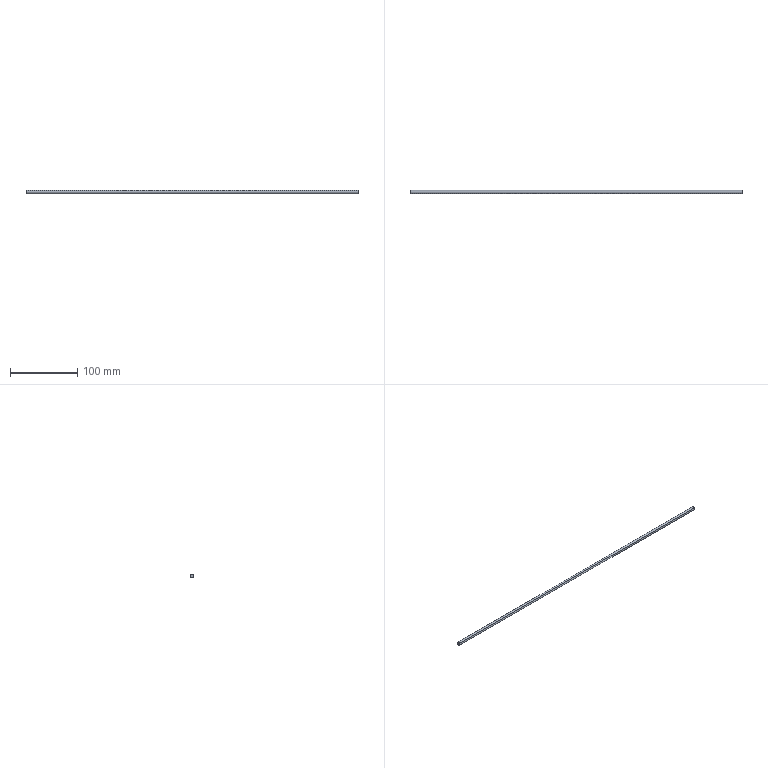Component | SolidWorks | SlideRod-2 | 1 solid | 4 faces | box 493.5 x 5 x 5 mm | volume 9690 mm3 | cylinder 2 | plane 2 | commonest cylinder face diameters 5 x2
build123d program:
from build123d import *

# Parameters (mm, degrees)
SKETCH1_R           = 2.5
BOSS_EXTRUDE1_DEPTH = 493.5


with BuildPart() as part:
    # Sketch1 → Boss-Extrude1 (new body)
    with BuildSketch(Plane(origin=(0, 0, 0), x_dir=(1, 0, 0), z_dir=(0, 1, 0))):
        with Locations(Location((0, 0, 0), (0, 0, 270))):
            Circle(SKETCH1_R)
    extrude(amount=BOSS_EXTRUDE1_DEPTH)


solid = part.part

# Placed as in the assembly
solid = solid.moved(Location((298.5, 220, -145), (0, 0, 90)))
STEP:
#1=CARTESIAN_POINT('',(11.752,8.735,-5.774));
#2=VERTEX_POINT('',#1);
#3=CARTESIAN_POINT('',(11.752,8.588,-5.643));
#4=VERTEX_POINT('',#3);
#5=CARTESIAN_POINT('',(11.752,8.661,-5.709));
#6=DIRECTION('',(1.,0.,0.));
#7=DIRECTION('',(0.,0.7491,-0.6624));
#8=AXIS2_PLACEMENT_3D('',#5,#6,#7);
#9=CIRCLE('',#8,0.09843);
#10=EDGE_CURVE('',#2,#4,#9,.T.);
#11=ORIENTED_EDGE('',*,*,#10,.F.);
#12=CARTESIAN_POINT('',(-7.677,8.735,-5.774));
#13=VERTEX_POINT('',#12);
#14=CARTESIAN_POINT('',(11.752,8.735,-5.774));
#15=DIRECTION('',(-1.,-0.,-0.));
#16=VECTOR('',#15,39.37);
#17=LINE('',#14,#16);
#18=EDGE_CURVE('',#2,#13,#17,.T.);
#19=ORIENTED_EDGE('',*,*,#18,.T.);
#20=CARTESIAN_POINT('',(-7.677,8.588,-5.643));
#21=VERTEX_POINT('',#20);
#22=CARTESIAN_POINT('',(-7.677,8.661,-5.709));
#23=DIRECTION('',(1.,0.,0.));
#24=DIRECTION('',(0.,0.7491,-0.6624));
#25=AXIS2_PLACEMENT_3D('',#22,#23,#24);
#26=CIRCLE('',#25,0.09843);
#27=EDGE_CURVE('',#13,#21,#26,.T.);
#28=ORIENTED_EDGE('',*,*,#27,.T.);
#29=CARTESIAN_POINT('',(11.752,8.588,-5.643));
#30=DIRECTION('',(-1.,-0.,-0.));
#31=VECTOR('',#30,39.37);
#32=LINE('',#29,#31);
#33=EDGE_CURVE('',#4,#21,#32,.T.);
#34=ORIENTED_EDGE('',*,*,#33,.F.);
#35=EDGE_LOOP('',(#11,#19,#28,#34));
#36=FACE_OUTER_BOUND('',#35,.T.);
#37=CARTESIAN_POINT('',(11.752,8.661,-5.709));
#38=DIRECTION('',(-1.,-0.,-0.));
#39=DIRECTION('',(0.,-0.7491,0.6624));
#40=AXIS2_PLACEMENT_3D('',#37,#38,#39);
#41=CYLINDRICAL_SURFACE('',#40,0.09843);
#42=ADVANCED_FACE('',(#36),#41,.T.);
#43=ORIENTED_EDGE('',*,*,#18,.F.);
#44=CARTESIAN_POINT('',(11.752,8.661,-5.709));
#45=DIRECTION('',(1.,0.,0.));
#46=DIRECTION('',(0.,0.7491,-0.6624));
#47=AXIS2_PLACEMENT_3D('',#44,#45,#46);
#48=CIRCLE('',#47,0.09843);
#49=EDGE_CURVE('',#4,#2,#48,.T.);
#50=ORIENTED_EDGE('',*,*,#49,.F.);
#51=ORIENTED_EDGE('',*,*,#33,.T.);
#52=CARTESIAN_POINT('',(-7.677,8.661,-5.709));
#53=DIRECTION('',(1.,0.,0.));
#54=DIRECTION('',(0.,0.7491,-0.6624));
#55=AXIS2_PLACEMENT_3D('',#52,#53,#54);
#56=CIRCLE('',#55,0.09843);
#57=EDGE_CURVE('',#21,#13,#56,.T.);
#58=ORIENTED_EDGE('',*,*,#57,.T.);
#59=EDGE_LOOP('',(#43,#50,#51,#58));
#60=FACE_OUTER_BOUND('',#59,.T.);
#61=CARTESIAN_POINT('',(11.752,8.661,-5.709));
#62=DIRECTION('',(-1.,-0.,-0.));
#63=DIRECTION('',(0.,-0.7491,0.6624));
#64=AXIS2_PLACEMENT_3D('',#61,#62,#63);
#65=CYLINDRICAL_SURFACE('',#64,0.09843);
#66=ADVANCED_FACE('',(#60),#65,.T.);
#67=ORIENTED_EDGE('',*,*,#49,.T.);
#68=ORIENTED_EDGE('',*,*,#10,.T.);
#69=EDGE_LOOP('',(#67,#68));
#70=FACE_OUTER_BOUND('',#69,.T.);
#71=CARTESIAN_POINT('',(11.752,8.661,-5.709));
#72=DIRECTION('',(1.,0.,0.));
#73=DIRECTION('',(-0.,0.7491,-0.6624));
#74=AXIS2_PLACEMENT_3D('',#71,#72,#73);
#75=PLANE('',#74);
#76=ADVANCED_FACE('',(#70),#75,.T.);
#77=ORIENTED_EDGE('',*,*,#57,.F.);
#78=ORIENTED_EDGE('',*,*,#27,.F.);
#79=EDGE_LOOP('',(#77,#78));
#80=FACE_OUTER_BOUND('',#79,.T.);
#81=CARTESIAN_POINT('',(-7.677,8.661,-5.709));
#82=DIRECTION('',(1.,0.,0.));
#83=DIRECTION('',(-0.,0.7491,-0.6624));
#84=AXIS2_PLACEMENT_3D('',#81,#82,#83);
#85=PLANE('',#84);
#86=ADVANCED_FACE('',(#80),#85,.F.);
#87=CLOSED_SHELL('',(#42,#66,#76,#86));
#88=MANIFOLD_SOLID_BREP('',#87);
#89=CARTESIAN_POINT('',(0.,0.,0.));
#90=DIRECTION('',(0.,0.,1.));
#91=DIRECTION('',(1.,0.,0.));
#92=AXIS2_PLACEMENT_3D('',#89,#90,#91);
#93=(LENGTH_UNIT()NAMED_UNIT(*)SI_UNIT($,.METRE.));
#94=LENGTH_MEASURE_WITH_UNIT(LENGTH_MEASURE(0.0254),#93);
#95=DIMENSIONAL_EXPONENTS(1.,0.,0.,0.,0.,0.,0.);
#96=(CONVERSION_BASED_UNIT('',#94)LENGTH_UNIT()NAMED_UNIT(#95));
#97=UNCERTAINTY_MEASURE_WITH_UNIT(LENGTH_MEASURE(0.00001),#96,'','');
#98=(NAMED_UNIT(*)PLANE_ANGLE_UNIT()SI_UNIT($,.RADIAN.));
#99=(NAMED_UNIT(*)SI_UNIT($,.STERADIAN.)SOLID_ANGLE_UNIT());
#100=(GEOMETRIC_REPRESENTATION_CONTEXT(3)GLOBAL_UNCERTAINTY_ASSIGNED_CONTEXT((#97))GLOBAL_UNIT_ASSIGNED_CONTEXT((#96,#98,#99))REPRESENTATION_CONTEXT('',''));
#101=ADVANCED_BREP_SHAPE_REPRESENTATION('',(#88,#92),#100);
#102=COLOUR_RGB('',0.7922,0.8196,0.9333);
#103=FILL_AREA_STYLE_COLOUR('',#102);
#104=FILL_AREA_STYLE('',(#103));
#105=SURFACE_STYLE_FILL_AREA(#104);
#106=SURFACE_SIDE_STYLE('',(#105));
#107=SURFACE_STYLE_USAGE(.BOTH.,#106);
#108=PRESENTATION_STYLE_ASSIGNMENT((#107));
#109=STYLED_ITEM('',(#108),#88);
#110=PRESENTATION_LAYER_ASSIGNMENT('','',(#109));
#111=(LENGTH_UNIT()NAMED_UNIT(*)SI_UNIT($,.METRE.));
#112=LENGTH_MEASURE_WITH_UNIT(LENGTH_MEASURE(0.0254),#111);
#113=DIMENSIONAL_EXPONENTS(1.,0.,0.,0.,0.,0.,0.);
#114=(CONVERSION_BASED_UNIT('',#112)LENGTH_UNIT()NAMED_UNIT(#113));
#115=UNCERTAINTY_MEASURE_WITH_UNIT(LENGTH_MEASURE(0.00001),#114,'','');
#116=(NAMED_UNIT(*)PLANE_ANGLE_UNIT()SI_UNIT($,.RADIAN.));
#117=(NAMED_UNIT(*)SI_UNIT($,.STERADIAN.)SOLID_ANGLE_UNIT());
#118=(GEOMETRIC_REPRESENTATION_CONTEXT(3)GLOBAL_UNCERTAINTY_ASSIGNED_CONTEXT((#115))GLOBAL_UNIT_ASSIGNED_CONTEXT((#114,#116,#117))REPRESENTATION_CONTEXT('',''));
#119=MECHANICAL_DESIGN_GEOMETRIC_PRESENTATION_REPRESENTATION('',(#109),#118);